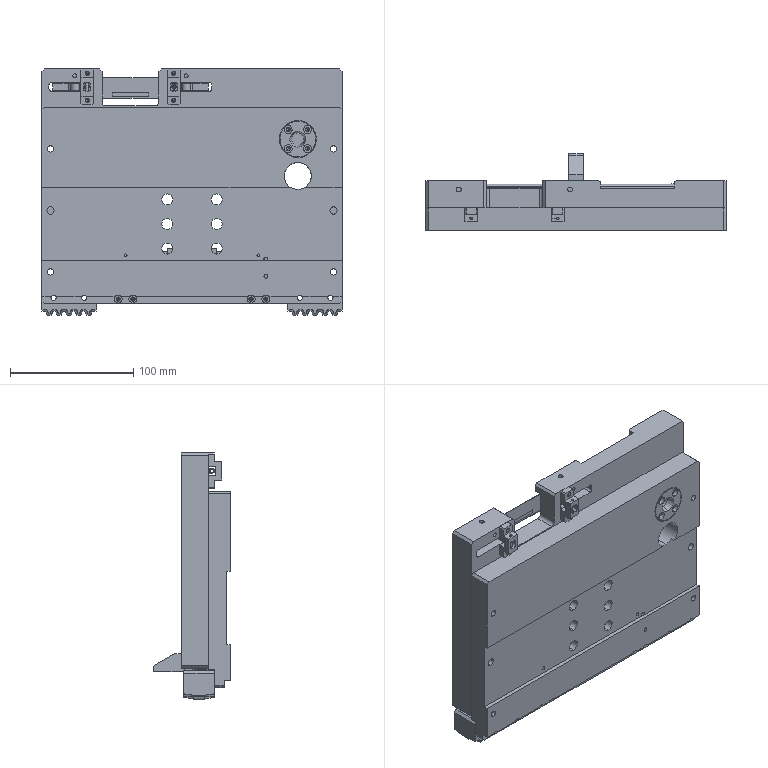Assembly | SolidWorks | mm | 23 component files | 23 solids | 1517 faces | box 244 x 62.5 x 200 mm | volume 1253407 mm3 | plane 683 | cylinder 528 | cone 168 | spline 134 | torus 4 | commonest cylinder face diameters 2.5 x60 3.4 x56 6.5 x52 3 x50 2 x45 4 x41 6 x29 15 x24
Bill of materials:
AdapterAluminumPlate | 1 | 6061 | Very thin flat rectangular sheet or plate with no visible holes or cutouts.
MAC22-D2-L14 | 1 | Steel Part | Solid round pin with a chamfer at both ends.
MGN9C | 2 |  | Rectangular block with a rectangular channel through its underside and semicircular grooves running along the channel walls. It has stepped side flanges and side grooves, and looks like a linear-guide carriage block body.
MGN9C1R55Z0C(E=7.5) | 2 |  | Short straight bar with chamfered corners and a semicircular groove along each side. Two round holes pass through it. It looks like a short section of profiled guide rail.
SAWH02-03101A0MountingPlate1 | 1 | 6061 | Thick rectangular plate with a step along one long edge and a pattern of through holes. The pattern includes six medium holes, two large holes near one corner (one ringed by a counterbore or recess with small holes around it) and several small holes near the edges.
SAWH02-03102A0MountingPlate2 | 1 | Light Green Fiberglass Board | Thick plate with a rectangular notch in the top edge and a wide rectangular cutout in the bottom edge, giving two lower legs. It has four medium holes in a square pattern, one large hole, corner holes, and a long slot in each of the two upper tabs.
SAWH02-03103A0SynchronousToothedMetalPart | 2 | SUS304 | Rectangular block with two long through slots and a row of evenly spaced rounded tooth-shaped notches along one edge. Some corners are chamfered.
SAWH02-03105A0MountingPlate5 | 2 | 6061 | Rectangular block with two rounded corners at one end. One large round bore passes through the top face, and two smaller holes are drilled into one side face.
SAWH02-03106A0MountingPlate6 | 1 | Polyurethane(Yellow) | Rectangular bar with two counterbored through holes spaced along its length.
SAWH02-03107A0MountingPlate7 | 1 | SKD11 | Stepped T-shaped block. A flat flange with chamfered corners has four through holes. A narrower projecting body has a sloping top surface that ends in a rounded nose.
SAWH02-03108A0MountingPlate8 | 1 | A6061 | Long rectangular bar with a recessed step in the middle of one long edge. Each end has four through holes in a 2x2 pattern. Two small holes sit on the recessed top surface, and the corners are chamfered.
SAWH02-03109A0RearPushBlock | 1 | Light Green Fiberglass Board | Long thin bar with two downward tabs, each with a long vertical slot. The ends are chamfered or rounded, and the tab roots have fillets.
SAWH02-03110A0StopBlock1 | 2 | SUS304 | Elongated rectangular bar with rounded ends. A cylindrical boss with a larger through-hole sticks out from one long side, blended into the bar with concave fillets. A smaller tab with a small through-hole sits next to it. Both hole axes are perpendicular to the bar's flat face.
SAWH02-03111A0TensionSpringMountingBlock | 2 | Q235A | Stepped, roughly prismatic block with an offset Z- or S-shaped side profile. It has chamfered corners. A rounded-rectangle (slot-like) opening goes through the middle. Two round holes go through near the ends, and smaller cross-holes run along other axes.
SAWH02-03112A0LocatingBlock | 1 | 45 | Flanged cylindrical bushing or nut-like part. A thin circular flange has four evenly spaced through-holes. A smaller cylindrical hub projects from one face. A central bore runs through the whole part, and the edges are chamfered.
YAUS-D4-L20 | 2 |  | Extension-spring-like part. The body is a simplified solid cylinder, not modelled coils, and it has an open circular hook loop at each end. Both hooks lie in the same plane and are offset to opposite sides of the axis.
Mates:
1. parallel | MGN9C1R55Z0C(E=7.5)-9 face at (77.01, -16.888, -89.292) dir (-1, 0, 0) | MGN9C1R55Z0C(E=7.5)-10 face at (-30.99, -16.888, -89.292) dir (-1, 0, 0)
2. coincident | MGN9C1R55Z0C(E=7.5)-9 face at (77.01, -20.388, -89.292) dir (0, -1, 0) | MGN9C1R55Z0C(E=7.5)-10 face at (-30.99, -20.388, -89.292) dir (0, -1, 0)
3. coincident | SAWH02-03101A0MountingPlate1-2 face at (27.51, -12.388, 21.208) dir (0, 1, 0) | SAWH02-03102A0MountingPlate2-1 face at (27.51, -12.388, -35.292) dir (0, -1, 0)
4. coincident | SAWH02-03109A0RearPushBlock-3 face at (27.51, -0.8876, -114.792) dir (0, -1, 0) | SAWH02-03108A0MountingPlate8-2 face at (27.51, -0.8876, -110.792) dir (0, 1, 0)
5. width | SAWH02-03109A0RearPushBlock-3 face at (125.51, 7.112, -101.792) dir (1, 0, 0) | SAWH02-03109A0RearPushBlock-3 face at (-70.49, 7.112, -101.792) dir (-1, 0, 0) | SAWH02-03108A0MountingPlate8-2 face at (-38.49, -0.8876, -95.792) dir (-1, 0, 0) | SAWH02-03108A0MountingPlate8-2 face at (93.51, -0.8876, -95.792) dir (1, 0, 0)
6. width | SAWH02-03102A0MountingPlate2-1 face at (-94.49, 9.612, 52.208) dir (-1, 0, 0) | SAWH02-03102A0MountingPlate2-1 face at (149.51, 9.612, 52.208) dir (1, 0, 0) | MGN9C1R55Z0C(E=7.5)-9 face at (86.01, -20.388, -89.292) dir (1, 0, 0) | MGN9C1R55Z0C(E=7.5)-10 face at (-30.99, -16.888, -89.292) dir (-1, 0, 0)
7. width | SAWH02-03102A0MountingPlate2-1 face at (102.51, -12.388, -122.792) dir (-1, 0, 0) | SAWH02-03102A0MountingPlate2-1 face at (-47.49, -12.388, -122.792) dir (1, 0, 0) | MGN9C1R55Z0C(E=7.5)-9 face at (86.01, -20.388, -89.292) dir (1, 0, 0) | MGN9C1R55Z0C(E=7.5)-10 face at (-30.99, -16.888, -89.292) dir (-1, 0, 0)
8. coincident | MGN9C1R55Z0C(E=7.5)-10 face at (-30.99, -20.388, -89.292) dir (0, -1, 0) | SAWH02-03105A0MountingPlate5-7 face at (93.51, -20.388, -130.792) dir (0, -1, 0)
9. coincident | SAWH02-03108A0MountingPlate8-2 face at (-38.49, -0.8876, -125.792) dir (0, 0, -1) | SAWH02-03107A0MountingPlate7-5 face at (41.51, 7.112, -125.792) dir (0, 0, -1)
10. width | SAWH02-03108A0MountingPlate8-2 face at (93.51, -0.8876, -95.792) dir (1, 0, 0) | SAWH02-03108A0MountingPlate8-2 face at (-38.49, -0.8876, -95.792) dir (-1, 0, 0) | SAWH02-03107A0MountingPlate7-5 face at (13.51, 7.112, -110.792) dir (-1, 0, 0) | SAWH02-03107A0MountingPlate7-5 face at (41.51, 7.112, -110.792) dir (1, 0, 0)
11. coincident | SAWH02-03101A0MountingPlate1-2 face at (-35.49, -20.388, -91.792) dir (0, 1, 0) | MGN9C1R55Z0C(E=7.5)-9 face at (82.31, -20.388, -89.292) dir (0, -1, 0)
12. coincident | MGN9C1R55Z0C(E=7.5)-9 face at (86.01, -13.888, -89.292) dir (0, 1, 0) | MGN9C-9 face at (86.01, -13.888, -83.292) dir (0, -1, 0)
13. width | MGN9C-9 face at (86.01, -20.388, -83.292) dir (-1, 0, 0) | MGN9C-9 face at (77.01, -16.888, -83.292) dir (1, 0, 0) | MGN9C1R55Z0C(E=7.5)-9 face at (86.01, -20.388, -89.292) dir (1, 0, 0) | MGN9C1R55Z0C(E=7.5)-9 face at (77.01, -16.888, -89.292) dir (-1, 0, 0)
14. coincident | SAWH02-03108A0MountingPlate8-2 face at (71.51, -11.888, -95.792) dir (1, 0, 0) | MGN9C-9 face at (71.51, -18.388, -96.342) dir (-1, 0, 0)
15. concentric | SAWH02-03108A0MountingPlate8-2 face at (74.01, -0.8876, -115.792) dir (0, 1, 0) r 1.7 | MGN9C-9 face at (74.01, -10.388, -115.792) dir (0, -1, 0) r 1.5
16. width | MGN9C-10 face at (-21.99, -20.388, -83.292) dir (-1, 0, 0) | MGN9C-10 face at (-30.99, -16.888, -83.292) dir (1, 0, 0) | MGN9C1R55Z0C(E=7.5)-10 face at (-21.99, -20.388, -89.292) dir (1, 0, 0) | MGN9C1R55Z0C(E=7.5)-10 face at (-30.99, -16.888, -89.292) dir (-1, 0, 0)
17. coincident | MGN9C1R55Z0C(E=7.5)-10 face at (-21.99, -13.888, -89.292) dir (0, 1, 0) | MGN9C-10 face at (-21.99, -13.888, -83.292) dir (0, -1, 0)
18. coincident | SAWH02-03108A0MountingPlate8-2 face at (-16.49, -11.888, -95.792) dir (-1, 0, 0) | MGN9C-10 face at (-16.49, -10.388, -96.342) dir (1, 0, 0)
19. concentric | SAWH02-03108A0MountingPlate8-2 face at (-18.99, -0.8876, -105.792) dir (0, 1, 0) r 1.7 | MGN9C-10 face at (-18.99, -10.388, -105.792) dir (0, -1, 0) r 1.5
20. coincident | SAWH02-03108A0MountingPlate8-2 face at (27.51, -10.388, -110.792) dir (0, -1, 0) | MGN9C-10 face at (-36.49, -10.388, -96.342) dir (0, 1, 0)
21. coincident | SAWH02-03108A0MountingPlate8-2 face at (27.51, -0.8876, -110.792) dir (0, 1, 0) | SAWH02-03107A0MountingPlate7-5 face at (27.51, -0.8876, -118.292) dir (0, -1, 0)
22. coincident | SAWH02-03102A0MountingPlate2-1 face at (128.01, 0.4124, 7.208) dir (0, 1, 0) | assembly face at (27.51, 0.4124, -37.792) dir (0, -1, 0)
23. coincident | SAWH02-03102A0MountingPlate2-1 face at (128.01, 0.4124, 7.208) dir (0, 1, 0) | assembly face at (27.51, 0.4124, -37.792) dir (0, -1, 0)
24. coincident | SAWH02-03102A0MountingPlate2-1 face at (16.51, -295.069, 26.208) dir (0, 0, -1) | assembly face at (134.01, 4.062, 26.208) dir (0, 0, 1)
25. width | SAWH02-03102A0MountingPlate2-1 face at (133.51, -295.069, -122.792) dir (-1, 0, 0) | SAWH02-03102A0MountingPlate2-1 face at (-78.49, -295.069, 21.208) dir (1, 0, 0) | assembly face at (-72.49, 7.412, 6.208) dir (-1, 0, 0) | assembly face at (127.51, 7.412, 6.208) dir (1, 0, 0)
26. width | SAWH02-03101A0MountingPlate1-2 face at (-94.49, -12.388, -138.792) dir (-1, 0, 0) | SAWH02-03101A0MountingPlate1-2 face at (149.51, -12.388, -138.792) dir (1, 0, 0) | SAWH02-03102A0MountingPlate2-1 face at (-94.49, 9.612, 52.208) dir (-1, 0, 0) | SAWH02-03102A0MountingPlate2-1 face at (149.51, 9.612, 52.208) dir (1, 0, 0)
27. coincident | SAWH02-03101A0MountingPlate1-2 face at (-94.49, -12.388, -138.792) dir (0, 0, -1) | SAWH02-03105A0MountingPlate5-7 face at (81.51, -10.388, -138.792) dir (0, 0, -1)
28. concentric | SAWH02-03102A0MountingPlate2-1 face at (-67.74, 2.612, 28.208) dir (0, 0, 1) r 2 | SAWH02-03110A0StopBlock1-1 face at (-67.74, 2.612, 40.708) dir (0, 0, -1) r 2
29. width | SAWH02-03102A0MountingPlate2-1 face at (-54.74, -12.388, 34.208) dir (0, 0, 1) | SAWH02-03102A0MountingPlate2-1 face at (-54.74, -12.388, 41.208) dir (0, 0, -1) | SAWH02-03110A0StopBlock1-1 face at (-57.74, 3.112, 40.708) dir (0, 0, 1) | SAWH02-03110A0StopBlock1-1 face at (-57.74, 3.112, 34.708) dir (0, 0, -1)
30. angle | SAWH02-03110A0StopBlock1-1 face at (-62.254, 4.212, 40.708) dir (0, -1, 0) | AdapterAluminumSheetCellAssembly-1/AdapterAluminumPlate-1 face at (-22.49, 4.212, 36.658) dir (0, 1, 0)
31. coincident | SAWH02-03110A0StopBlock1-1 face at (-57.74, 3.112, 40.708) dir (0, 0, 1) | SAWH02-03110A0StopBlock1-2 face at (12.76, 3.112, 40.708) dir (0, 0, 1)
32. concentric | SAWH02-03102A0MountingPlate2-1 face at (22.76, 2.612, 28.208) dir (0, 0, 1) r 2 | SAWH02-03110A0StopBlock1-2 face at (22.76, 2.612, 34.708) dir (0, 0, 1) r 2
33. width | SAWH02-03110A0StopBlock1-1 face at (-49.74, 4.212, 40.708) dir (1, 0, 0) | SAWH02-03110A0StopBlock1-2 face at (4.76, 4.212, 34.708) dir (-1, 0, 0) | SAWH02-03102A0MountingPlate2-1 face at (-45.49, -12.388, 52.208) dir (1, 0, 0) | SAWH02-03102A0MountingPlate2-1 face at (0.5102, -12.388, 52.208) dir (-1, 0, 0)
34. coincident | SAWH02-03106A0MountingPlate6-8 face at (27.51, -6.388, -100.792) dir (0, 0, -1) | SAWH02-03108A0MountingPlate8-2 face at (7.41, -11.888, -100.792) dir (0, 0, 1)
35. coincident | SAWH02-03106A0MountingPlate6-8 face at (7.51, -11.888, -93.792) dir (0, -1, 0) | SAWH02-03108A0MountingPlate8-2 face at (27.51, -11.888, -110.792) dir (0, -1, 0)
36. concentric | SAWH02-03101A0MountingPlate1-2 face at (-87.49, -12.388, -112.792) dir (0, 1, 0) r 2.5 | SAWH02-03102A0MountingPlate2-1 face at (-87.49, 9.612, -112.792) dir (0, 1, 0) r 3.3
37. distance | MGN9C1R55Z0C(E=7.5)-9 face at (82.01, -20.388, -89.292) dir (0, 0, 1) | SAWH02-03101A0MountingPlate1-2 face at (-35.49, -20.388, -88.792) dir (0, 0, -1)
38. width | SAWH02-03111A0TensionSpringMountingBlock-1 face at (-57.74, -23.388, 52.208) dir (0, 0, 1) | SAWH02-03111A0TensionSpringMountingBlock-1 face at (-57.74, -23.388, 23.208) dir (0, 0, -1) | SAWH02-03102A0MountingPlate2-1 face at (-54.74, -12.388, 34.208) dir (0, 0, 1) | SAWH02-03102A0MountingPlate2-1 face at (-54.74, -12.388, 41.208) dir (0, 0, -1)
39. coincident | SAWH02-03102A0MountingPlate2-1 face at (27.51, -12.388, -35.292) dir (0, -1, 0) | SAWH02-03111A0TensionSpringMountingBlock-1 face at (-62.74, -12.388, 52.208) dir (0, 1, 0)
40. coincident | SAWH02-03102A0MountingPlate2-1 face at (-52.74, -12.388, 36.208) dir (-1, 0, 0) | SAWH02-03111A0TensionSpringMountingBlock-1 face at (-52.74, -23.388, 52.208) dir (1, 0, 0)
41. coincident | SAWH02-03102A0MountingPlate2-1 face at (27.51, -12.388, -35.292) dir (0, -1, 0) | SAWH02-03111A0TensionSpringMountingBlock-2 face at (17.76, -12.388, 23.208) dir (0, 1, 0)
42. coincident | SAWH02-03111A0TensionSpringMountingBlock-1 face at (-57.74, -23.388, 52.208) dir (0, 0, 1) | SAWH02-03111A0TensionSpringMountingBlock-2 face at (12.76, -23.388, 52.208) dir (0, 0, 1)
43. coincident | SAWH02-03102A0MountingPlate2-1 face at (7.76, -12.388, 36.208) dir (1, 0, 0) | SAWH02-03111A0TensionSpringMountingBlock-2 face at (7.76, -23.388, 23.208) dir (-1, 0, 0)
44. concentric | SAWH02-03110A0StopBlock1-1 face at (-57.74, 3.112, 40.708) dir (0, 0, -1) r 0.75 | YAUS-D4-L20-1 axis at (-57.74, 3.112, 37.708) dir (0, 0, 1)
45. width | SAWH02-03110A0StopBlock1-1 face at (-57.74, 3.112, 40.708) dir (0, 0, 1) | SAWH02-03110A0StopBlock1-1 face at (-57.74, 3.112, 34.708) dir (0, 0, -1) | YAUS-D4-L20-1 face at (-58.107, -13.884, 37.708) dir (0.0216, 0.9998, 0) r 2
46. concentric | SAWH02-03110A0StopBlock1-2 face at (12.76, 3.112, 34.708) dir (0, 0, 1) r 0.75 | YAUS-D4-L20-2 axis at (12.76, 3.112, 37.708) dir (0, 0, 1)
47. width | SAWH02-03110A0StopBlock1-2 face at (12.76, 3.112, 40.708) dir (0, 0, 1) | SAWH02-03110A0StopBlock1-2 face at (12.76, 3.112, 34.708) dir (0, 0, -1) | YAUS-D4-L20-2 face at (12.98, -13.886, 37.708) dir (-0.01292, 0.9999, 0) r 2
48. concentric | SAWH02-03111A0TensionSpringMountingBlock-1 face at (-57.74, -20.888, 23.208) dir (0, 0, 1) r 1 | MAC22-D2-L14-1 face at (-57.74, -20.888, 31.208) dir (0, 0, 1) r 1
49. coincident | SAWH02-03111A0TensionSpringMountingBlock-1 face at (-52.74, -17.388, 45.208) dir (0, 0, 1) | MAC22-D2-L14-1 face at (-57.74, -20.888, 45.208) dir (0, 0, 1)
50. coincident | SAWH02-03101A0MountingPlate1-2 face at (-94.49, -12.388, -138.792) dir (-1, 0, 0) | SAWH02-03103A0SynchronousToothedMetalPart-3 face at (-94.49, -17.388, -144.792) dir (-1, 0, 0)
51. coincident | SAWH02-03101A0MountingPlate1-2 face at (149.51, -12.388, -138.792) dir (1, 0, 0) | SAWH02-03103A0SynchronousToothedMetalPart-1 face at (149.51, -17.388, -144.792) dir (1, 0, 0)
52. coincident | SAWH02-03103A0SynchronousToothedMetalPart-1 face at (127.51, -4.888, -124.792) dir (0, 0, 1) | SAWH02-03103A0SynchronousToothedMetalPart-3 face at (-72.49, -4.888, -124.792) dir (0, 0, 1)
53. coincident | SAWH02-03101A0MountingPlate1-2 face at (149.51, -12.388, -138.792) dir (1, 0, 0) | SAWH02-03103A0SynchronousToothedMetalPart-1 face at (149.51, -17.388, -144.792) dir (1, 0, 0)
54. coincident | SAWH02-03101A0MountingPlate1-2 face at (27.51, -17.388, 21.208) dir (0, 1, 0) | SAWH02-03103A0SynchronousToothedMetalPart-1 face at (149.51, -17.388, -144.792) dir (0, -1, 0)
55. distance | SAWH02-03103A0SynchronousToothedMetalPart-1 face at (127.51, -4.888, -144.792) dir (0, 0, -1) | SAWH02-03101A0MountingPlate1-2 face at (-94.49, -12.388, -138.792) dir (0, 0, -1)
56. coincident | SAWH02-03101A0MountingPlate1-2 face at (93.51, -20.388, -91.792) dir (-1, 0, 0) | SAWH02-03105A0MountingPlate5-7 face at (93.51, -20.388, -130.792) dir (1, 0, 0)
57. coincident | SAWH02-03105A0MountingPlate5-7 face at (93.51, -0.3876, -130.792) dir (0, 1, 0) | SAWH02-03105A0MountingPlate5-8 face at (-14.49, -0.3876, -130.792) dir (0, 1, 0)
58. coincident | SAWH02-03101A0MountingPlate1-2 face at (-94.49, -12.388, -138.792) dir (0, 0, -1) | SAWH02-03105A0MountingPlate5-8 face at (-26.49, -10.388, -138.792) dir (0, 0, -1)
59. coincident | SAWH02-03101A0MountingPlate1-2 face at (-38.49, -20.388, -91.792) dir (1, 0, 0) | SAWH02-03105A0MountingPlate5-8 face at (-38.49, -20.388, -130.792) dir (-1, 0, 0)
60. coincident | SAWH02-03101A0MountingPlate1-2 face at (27.51, -17.388, 21.208) dir (0, 1, 0) | SAWH02-03103A0SynchronousToothedMetalPart-3 face at (-50.49, -17.388, -144.792) dir (0, -1, 0)
61. concentric | SAWH02-03101A0MountingPlate1-2 face at (113.51, -12.388, -4.792) dir (0, -1, 0) r 7.5 | SAWH02-03112A0LocatingBlock-1 face at (113.51, -30.388, -4.792) dir (0, -1, 0) r 7.5
62. coincident | SAWH02-03101A0MountingPlate1-2 face at (113.51, -25.388, -4.792) dir (0, -1, 0) | SAWH02-03112A0LocatingBlock-1 face at (128.51, -25.388, -4.792) dir (0, 1, 0)
63. parallel | SAWH02-03101A0MountingPlate1-2 face at (149.51, -12.388, -138.792) dir (1, 0, 0) | SAWH02-03112A0LocatingBlock-1 plane at (113.51, -30.388, -4.792) dir (1, 0, 0)
64. concentric | SAWH02-03106A0MountingPlate6-8 face at (17.51, -6.388, -93.792) dir (0, 0, 1) r 1.6 | SAWH02-03108A0MountingPlate8-2 face at (17.51, -6.388, -100.792) dir (0, 0, 1) r 1.25
65. concentric | SAWH02-03108A0MountingPlate8-2 face at (62.51, -0.8876, -121.792) dir (0, 1, 0) r 1.25 | SAWH02-03109A0RearPushBlock-3 face at (62.51, -2.888, -121.792) dir (0, 1, 0) r 1.6
66. coincident | SAWH02-03109A0RearPushBlock-3 face at (-70.49, 7.112, -101.792) dir (0, 0, 1) | assembly face at (134.01, 4.062, -101.792) dir (0, 0, -1)
67. coincident | MGN9C1R55Z0C(E=7.5)-9 face at (82.01, -20.388, -89.292) dir (0, 0, 1) | MGN9C1R55Z0C(E=7.5)-10 face at (-25.99, -20.388, -89.292) dir (0, 0, 1)